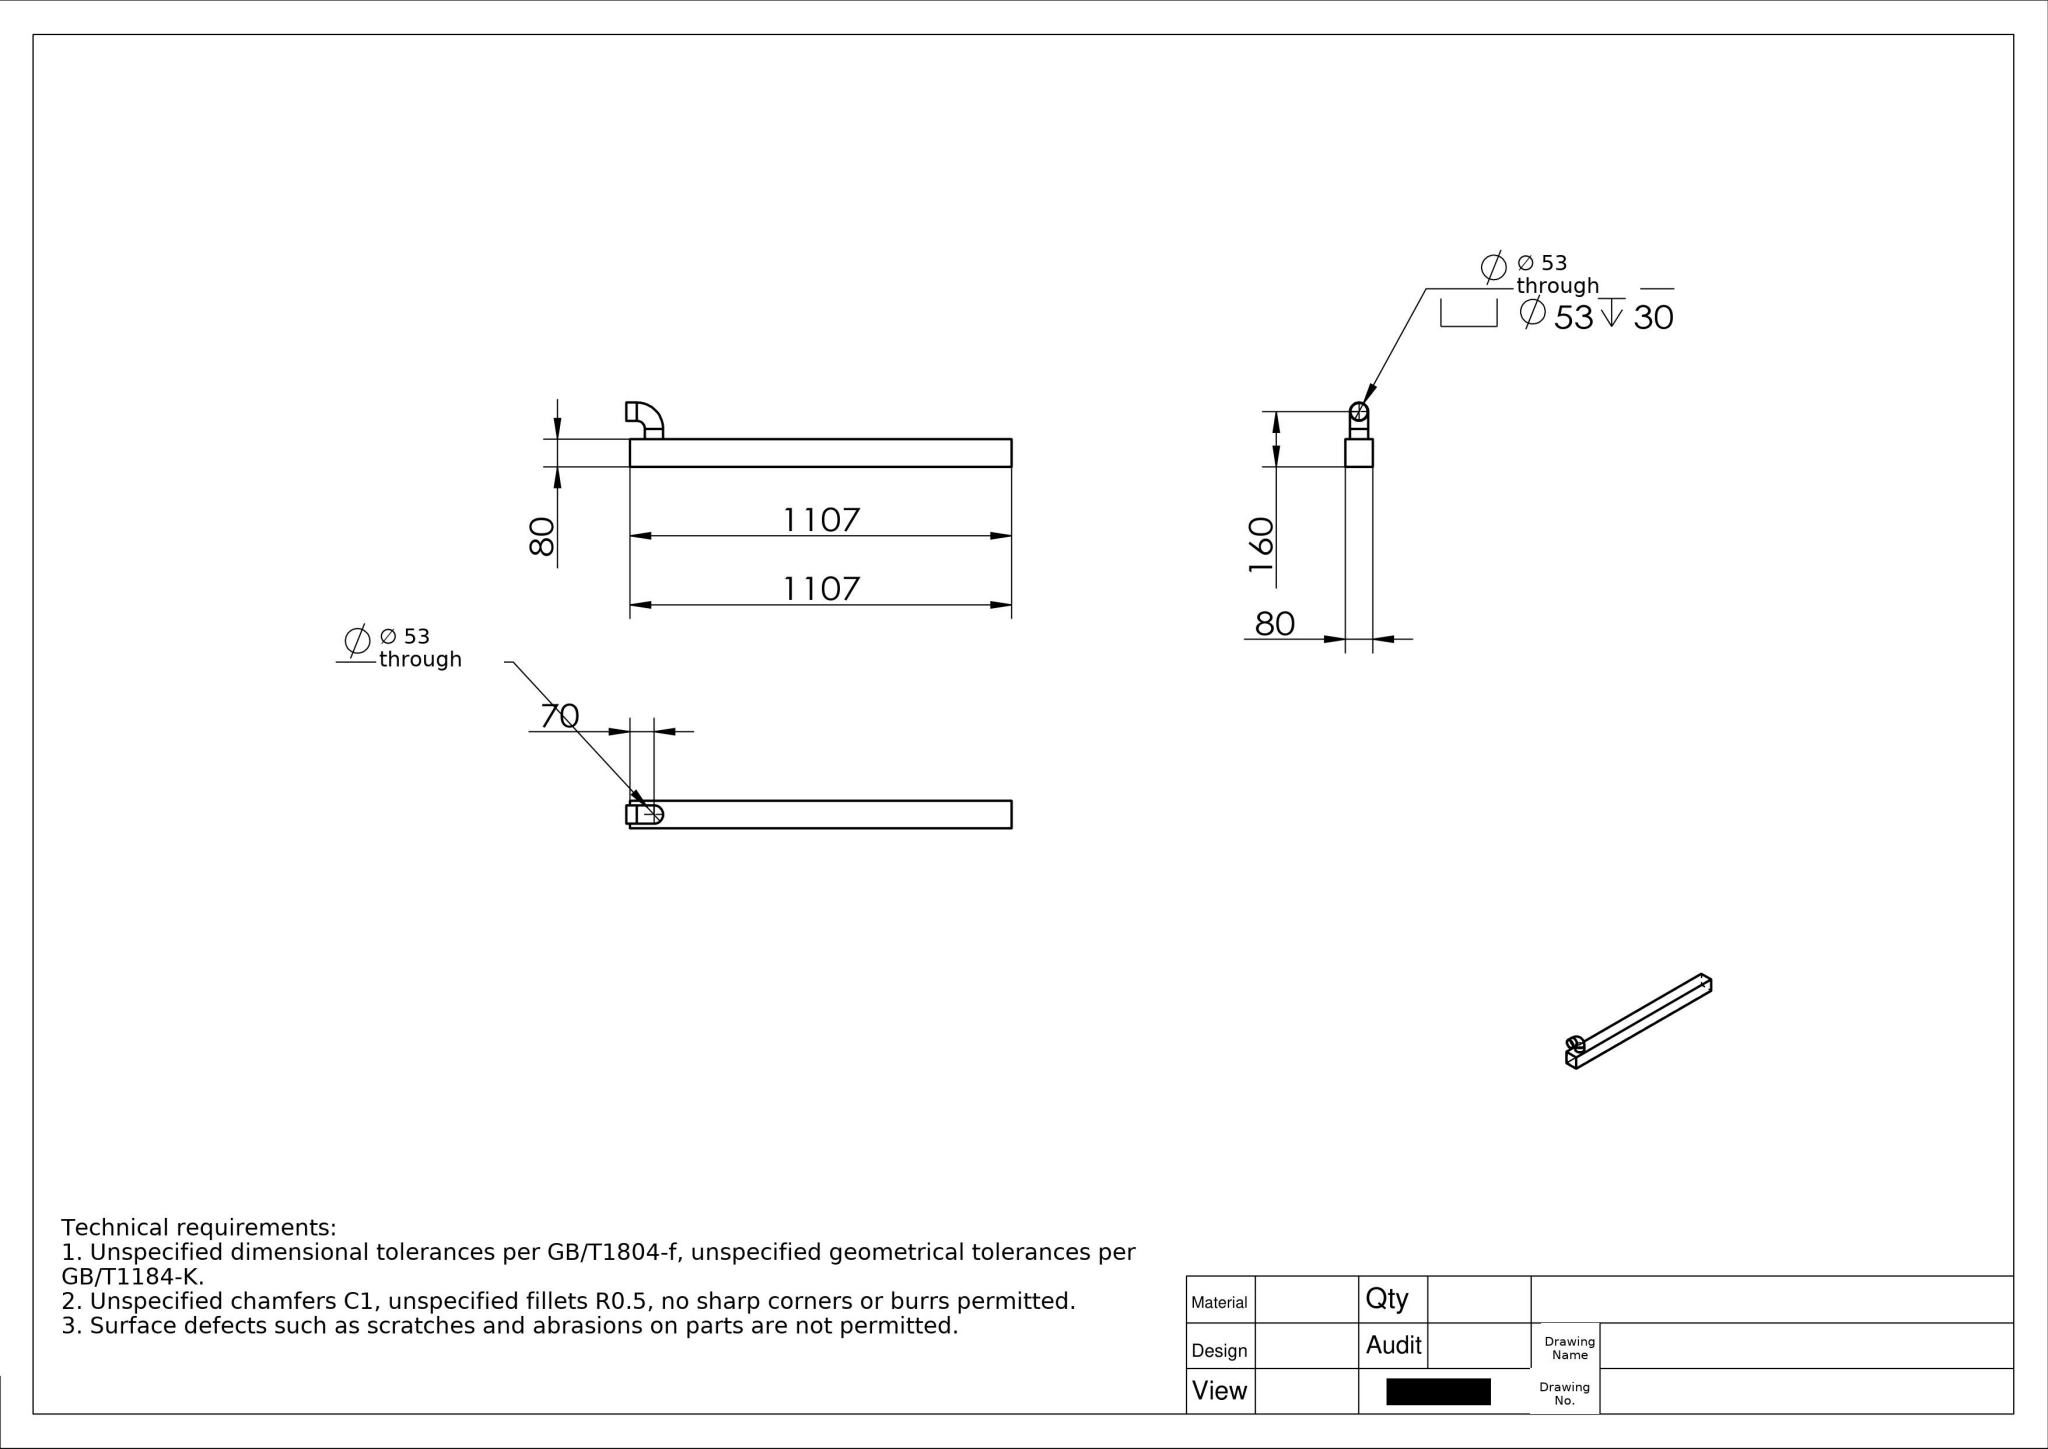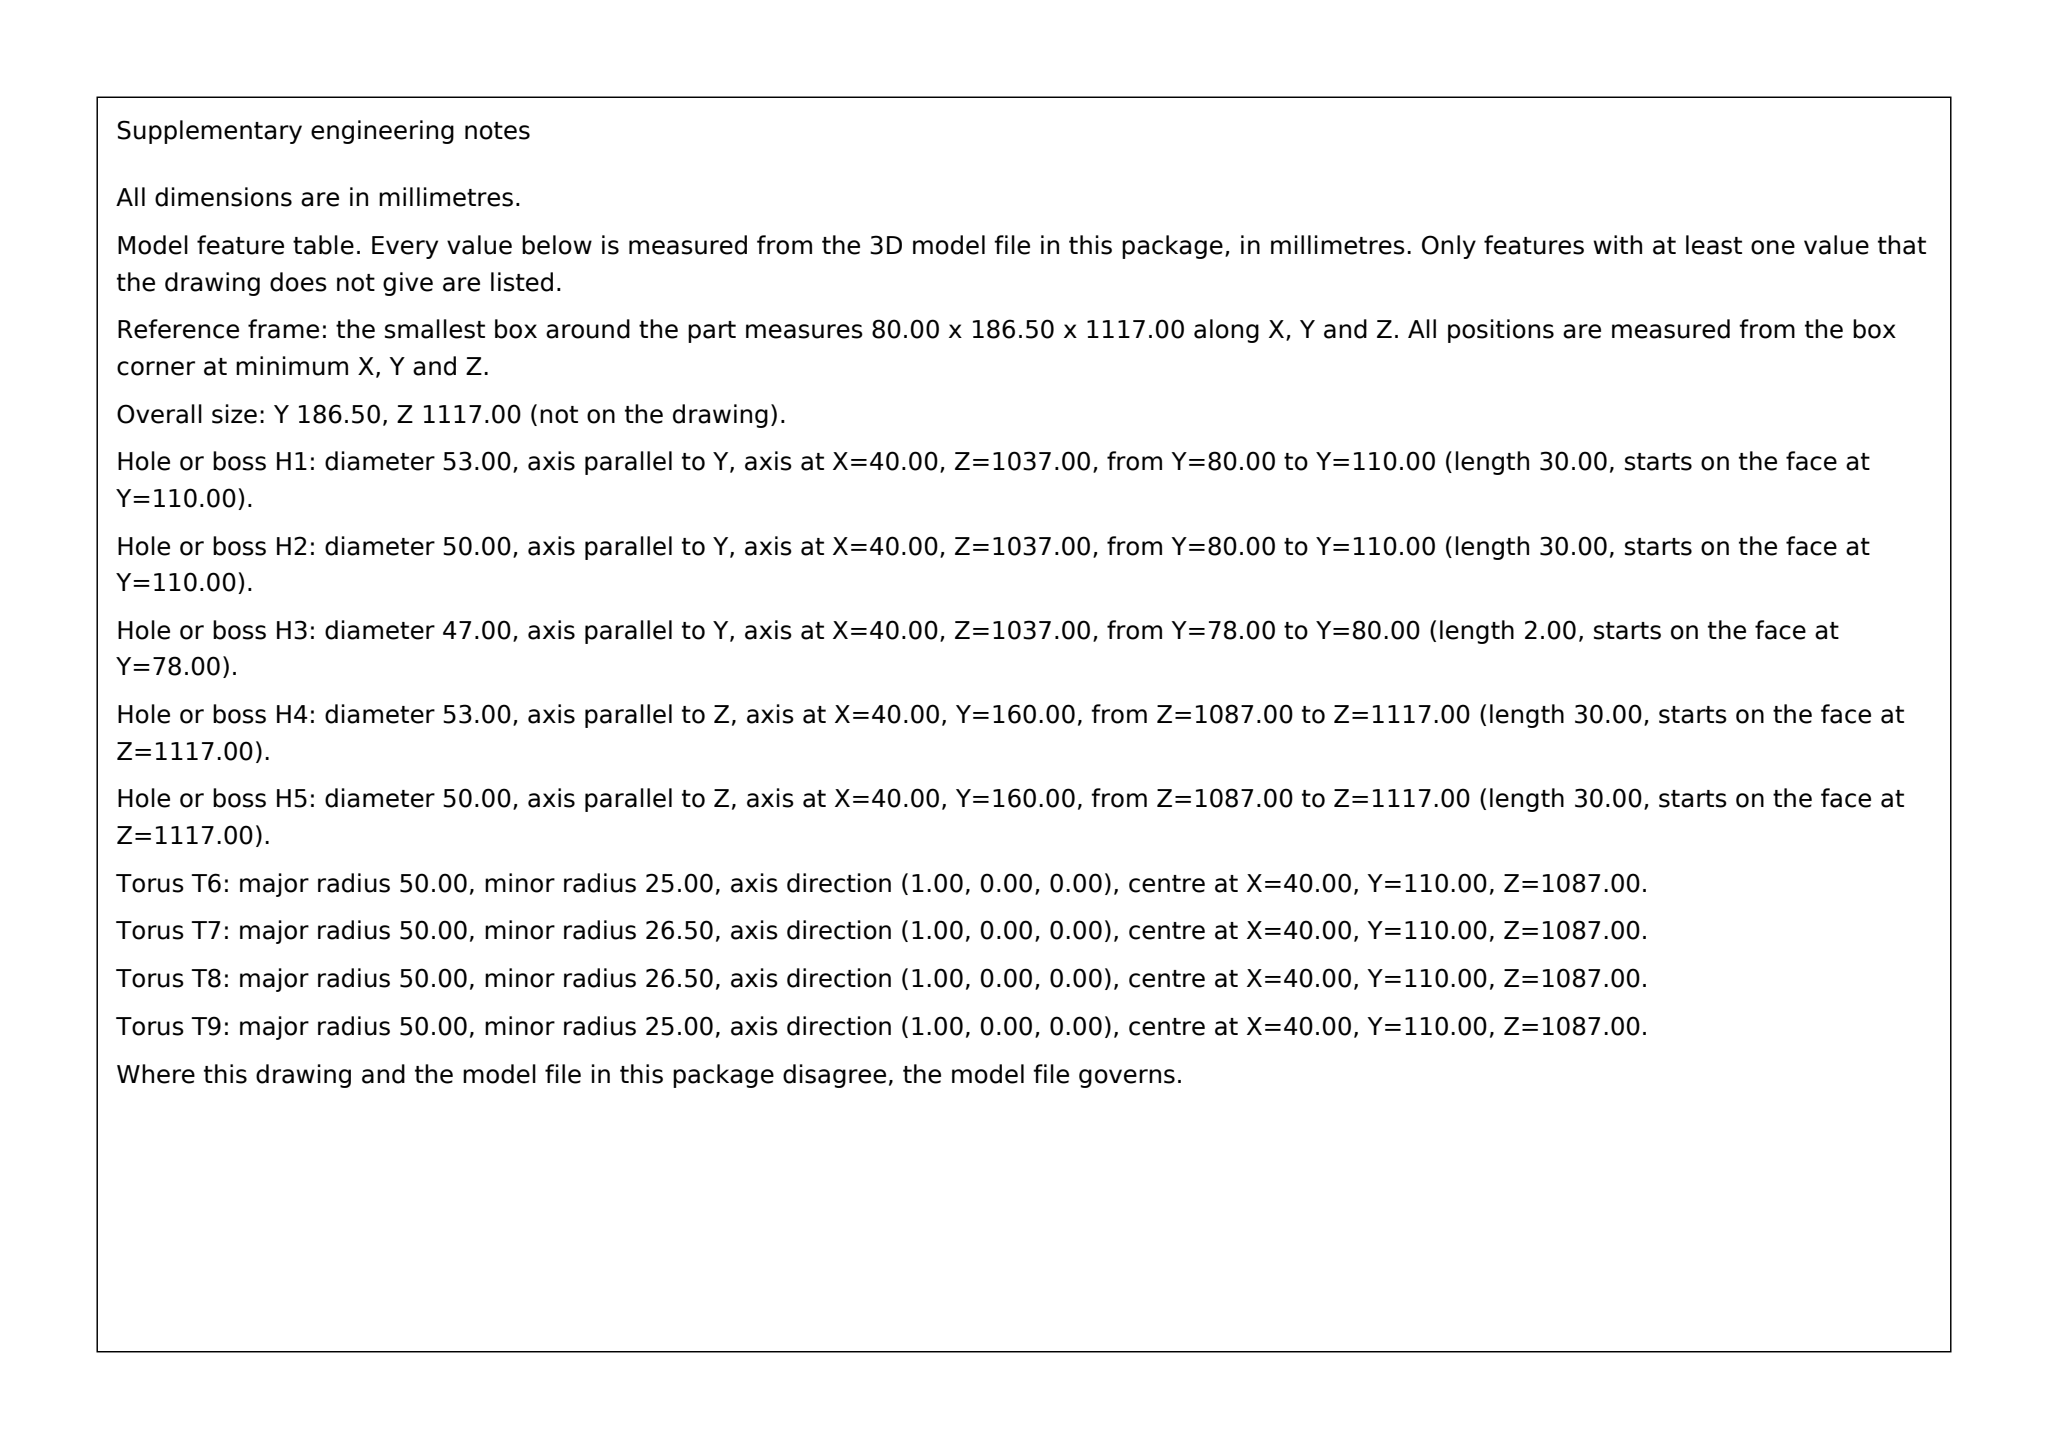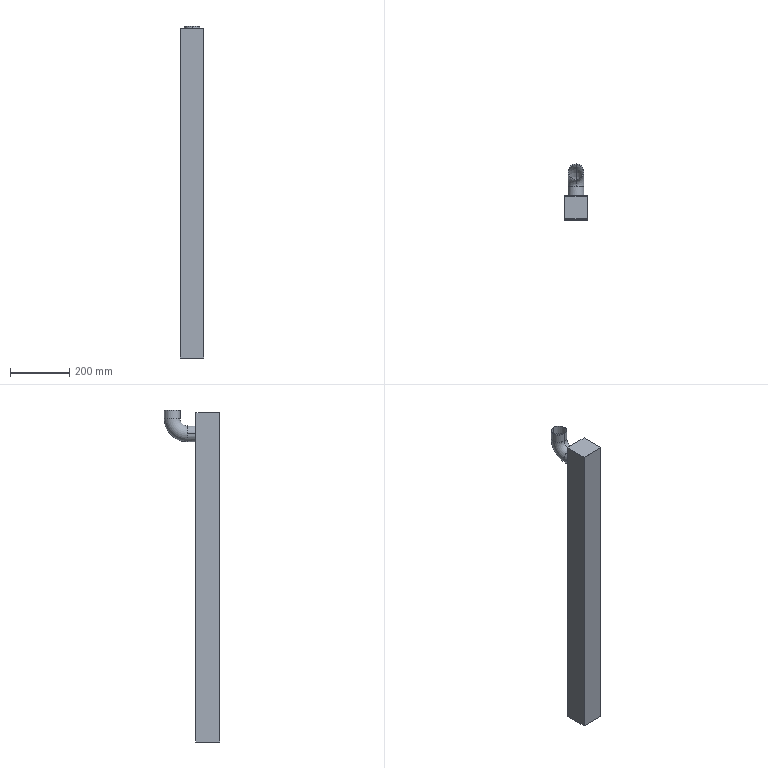Part | SolidWorks | mm | 1 solid | 27 faces | box 80 x 186.5 x 1117 mm | volume 738248 mm3 | plane 13 | cylinder 10 | torus 4 | commonest cylinder face diameters 50 x4 53 x4 47 x2
build123d program:
from build123d import *

# Parameters (mm, degrees)
SKETCH1_W                   = 80
SKETCH1_H                   = 80
SKETCH1_W_2                 = 76
SKETCH1_H_2                 = 76
BOSS_EXTRUDE1_DEPTH         = 1107
SKETCH2_W                   = 76
SKETCH2_H                   = 76
BOSS_EXTRUDE2_DEPTH         = 3
SKETCH3_R                   = 23.5
CUT_EXTRUDE1_DEPTH          = 10
SCAN_THIN_PART1_PROFILE_R   = 26.5
SCAN_THIN_PART1_PROFILE_R_2 = 25


with BuildPart() as part:
    # Sketch1 → Boss-Extrude1 (new body)
    with BuildSketch(Plane.XY):
        Rectangle(SKETCH1_W, SKETCH1_H)
        Rectangle(SKETCH1_W_2, SKETCH1_H_2, mode=Mode.SUBTRACT)
    extrude(amount=BOSS_EXTRUDE1_DEPTH)

    # Sketch2 → Boss-Extrude2 (add)
    with BuildSketch(Plane.XY.offset(1107)):
        Rectangle(SKETCH2_W, SKETCH2_H)
    extrude(amount=-BOSS_EXTRUDE2_DEPTH)

    # Sketch3 → Cut-Extrude1 (cut)
    with BuildSketch(Plane(origin=(0, 40, 0), x_dir=(1, 0, 0), z_dir=(0, 1, 0))):
        with Locations(Location((0, -1037, 0), (0, 0, 270))):
            Circle(SKETCH3_R)
    extrude(amount=-CUT_EXTRUDE1_DEPTH, mode=Mode.SUBTRACT)

    # Scan-Thin Part1: sweep along a path in Sketch4
    with BuildLine(Plane(origin=(0, 0, 0), x_dir=(0, 0, -1), z_dir=(1, 0, 0))) as scan_thin_part1_path:
        Line((-1037, 40), (-1037, 70))
        ThreePointArc((-1037, 70), (-1051.645, 105.355), (-1087, 120))
        Line((-1087, 120), (-1117, 120))
    # Scan-Thin Part1 profile (on start of the path) → Scan-Thin Part1 (sweep)
    with BuildSketch(Plane(origin=(0, 40, 1037), x_dir=(1, 0, 0), z_dir=(0, 1, 0))):
        Circle(SCAN_THIN_PART1_PROFILE_R)
        Circle(SCAN_THIN_PART1_PROFILE_R_2, mode=Mode.SUBTRACT)
    sweep(path=scan_thin_part1_path.line)


solid = part.part
STEP:
#1=CARTESIAN_POINT('',(-25.,70.,1037.));
#2=VERTEX_POINT('',#1);
#3=CARTESIAN_POINT('',(-0.,70.,1012.));
#4=VERTEX_POINT('',#3);
#5=CARTESIAN_POINT('',(-0.,70.,1037.));
#6=DIRECTION('',(0.,-1.,0.));
#7=DIRECTION('',(-1.,0.,0.));
#8=AXIS2_PLACEMENT_3D('',#5,#6,#7);
#9=CIRCLE('',#8,25.);
#10=EDGE_CURVE('',#2,#4,#9,.T.);
#11=ORIENTED_EDGE('',*,*,#10,.T.);
#12=CARTESIAN_POINT('',(-0.,145.,1087.));
#13=VERTEX_POINT('',#12);
#14=CARTESIAN_POINT('',(-0.,70.,1087.));
#15=DIRECTION('',(1.,0.,0.));
#16=DIRECTION('',(-0.,1.,0.));
#17=AXIS2_PLACEMENT_3D('',#14,#15,#16);
#18=CIRCLE('',#17,75.);
#19=EDGE_CURVE('',#4,#13,#18,.T.);
#20=ORIENTED_EDGE('',*,*,#19,.T.);
#21=CARTESIAN_POINT('',(-0.,95.,1087.));
#22=VERTEX_POINT('',#21);
#23=CARTESIAN_POINT('',(-0.,120.,1087.));
#24=DIRECTION('',(0.,0.,-1.));
#25=DIRECTION('',(-1.,0.,0.));
#26=AXIS2_PLACEMENT_3D('',#23,#24,#25);
#27=CIRCLE('',#26,25.);
#28=EDGE_CURVE('',#22,#13,#27,.T.);
#29=ORIENTED_EDGE('',*,*,#28,.F.);
#30=CARTESIAN_POINT('',(-0.,70.,1062.));
#31=VERTEX_POINT('',#30);
#32=CARTESIAN_POINT('',(-0.,70.,1087.));
#33=DIRECTION('',(1.,0.,0.));
#34=DIRECTION('',(-0.,1.,0.));
#35=AXIS2_PLACEMENT_3D('',#32,#33,#34);
#36=CIRCLE('',#35,25.);
#37=EDGE_CURVE('',#31,#22,#36,.T.);
#38=ORIENTED_EDGE('',*,*,#37,.F.);
#39=CARTESIAN_POINT('',(-0.,70.,1037.));
#40=DIRECTION('',(0.,-1.,0.));
#41=DIRECTION('',(-1.,0.,0.));
#42=AXIS2_PLACEMENT_3D('',#39,#40,#41);
#43=CIRCLE('',#42,25.);
#44=EDGE_CURVE('',#31,#2,#43,.T.);
#45=ORIENTED_EDGE('',*,*,#44,.T.);
#46=EDGE_LOOP('',(#11,#20,#29,#38,#45));
#47=FACE_OUTER_BOUND('',#46,.T.);
#48=CARTESIAN_POINT('',(-0.,70.,1087.));
#49=DIRECTION('',(1.,0.,0.));
#50=DIRECTION('',(-0.,1.,0.));
#51=AXIS2_PLACEMENT_3D('',#48,#49,#50);
#52=TOROIDAL_SURFACE('',#51,50.,25.);
#53=ADVANCED_FACE('',(#47),#52,.F.);
#54=CARTESIAN_POINT('',(-0.,70.,1010.5));
#55=VERTEX_POINT('',#54);
#56=CARTESIAN_POINT('',(26.5,70.,1037.));
#57=VERTEX_POINT('',#56);
#58=CARTESIAN_POINT('',(-0.,70.,1037.));
#59=DIRECTION('',(0.,-1.,0.));
#60=DIRECTION('',(-1.,0.,0.));
#61=AXIS2_PLACEMENT_3D('',#58,#59,#60);
#62=CIRCLE('',#61,26.5);
#63=EDGE_CURVE('',#55,#57,#62,.T.);
#64=ORIENTED_EDGE('',*,*,#63,.F.);
#65=CARTESIAN_POINT('',(-0.,146.5,1087.));
#66=VERTEX_POINT('',#65);
#67=CARTESIAN_POINT('',(-0.,70.,1087.));
#68=DIRECTION('',(1.,0.,0.));
#69=DIRECTION('',(-0.,1.,0.));
#70=AXIS2_PLACEMENT_3D('',#67,#68,#69);
#71=CIRCLE('',#70,76.5);
#72=EDGE_CURVE('',#55,#66,#71,.T.);
#73=ORIENTED_EDGE('',*,*,#72,.T.);
#74=CARTESIAN_POINT('',(-0.,93.5,1087.));
#75=VERTEX_POINT('',#74);
#76=CARTESIAN_POINT('',(-0.,120.,1087.));
#77=DIRECTION('',(0.,0.,-1.));
#78=DIRECTION('',(-1.,0.,0.));
#79=AXIS2_PLACEMENT_3D('',#76,#77,#78);
#80=CIRCLE('',#79,26.5);
#81=EDGE_CURVE('',#66,#75,#80,.T.);
#82=ORIENTED_EDGE('',*,*,#81,.T.);
#83=CARTESIAN_POINT('',(-0.,70.,1063.5));
#84=VERTEX_POINT('',#83);
#85=CARTESIAN_POINT('',(-0.,70.,1087.));
#86=DIRECTION('',(1.,0.,0.));
#87=DIRECTION('',(-0.,1.,0.));
#88=AXIS2_PLACEMENT_3D('',#85,#86,#87);
#89=CIRCLE('',#88,23.5);
#90=EDGE_CURVE('',#84,#75,#89,.T.);
#91=ORIENTED_EDGE('',*,*,#90,.F.);
#92=CARTESIAN_POINT('',(-0.,70.,1037.));
#93=DIRECTION('',(0.,-1.,0.));
#94=DIRECTION('',(-1.,0.,0.));
#95=AXIS2_PLACEMENT_3D('',#92,#93,#94);
#96=CIRCLE('',#95,26.5);
#97=EDGE_CURVE('',#57,#84,#96,.T.);
#98=ORIENTED_EDGE('',*,*,#97,.F.);
#99=EDGE_LOOP('',(#64,#73,#82,#91,#98));
#100=FACE_OUTER_BOUND('',#99,.T.);
#101=CARTESIAN_POINT('',(-0.,70.,1087.));
#102=DIRECTION('',(1.,0.,0.));
#103=DIRECTION('',(-0.,1.,0.));
#104=AXIS2_PLACEMENT_3D('',#101,#102,#103);
#105=TOROIDAL_SURFACE('',#104,50.,26.5);
#106=ADVANCED_FACE('',(#100),#105,.T.);
#107=ORIENTED_EDGE('',*,*,#28,.T.);
#108=CARTESIAN_POINT('',(-0.,145.,1117.));
#109=VERTEX_POINT('',#108);
#110=CARTESIAN_POINT('',(-0.,145.,1087.));
#111=DIRECTION('',(0.,-0.,1.));
#112=VECTOR('',#111,1000.);
#113=LINE('',#110,#112);
#114=EDGE_CURVE('',#13,#109,#113,.T.);
#115=ORIENTED_EDGE('',*,*,#114,.T.);
#116=CARTESIAN_POINT('',(-0.,95.,1117.));
#117=VERTEX_POINT('',#116);
#118=CARTESIAN_POINT('',(-0.,120.,1117.));
#119=DIRECTION('',(0.,0.,-1.));
#120=DIRECTION('',(-1.,0.,0.));
#121=AXIS2_PLACEMENT_3D('',#118,#119,#120);
#122=CIRCLE('',#121,25.);
#123=EDGE_CURVE('',#117,#109,#122,.T.);
#124=ORIENTED_EDGE('',*,*,#123,.F.);
#125=CARTESIAN_POINT('',(-0.,95.,1087.));
#126=DIRECTION('',(0.,-0.,1.));
#127=VECTOR('',#126,1000.);
#128=LINE('',#125,#127);
#129=EDGE_CURVE('',#22,#117,#128,.T.);
#130=ORIENTED_EDGE('',*,*,#129,.F.);
#131=EDGE_LOOP('',(#107,#115,#124,#130));
#132=FACE_OUTER_BOUND('',#131,.T.);
#133=CARTESIAN_POINT('',(-0.,120.,1087.));
#134=DIRECTION('',(0.,-0.,1.));
#135=DIRECTION('',(0.,-1.,0.));
#136=AXIS2_PLACEMENT_3D('',#133,#134,#135);
#137=CYLINDRICAL_SURFACE('',#136,25.);
#138=ADVANCED_FACE('',(#132),#137,.F.);
#139=CARTESIAN_POINT('',(-25.,40.,1037.));
#140=VERTEX_POINT('',#139);
#141=CARTESIAN_POINT('',(25.,40.,1037.));
#142=VERTEX_POINT('',#141);
#143=CARTESIAN_POINT('',(-0.,40.,1037.));
#144=DIRECTION('',(0.,-1.,0.));
#145=DIRECTION('',(-1.,-0.,0.));
#146=AXIS2_PLACEMENT_3D('',#143,#144,#145);
#147=CIRCLE('',#146,25.);
#148=EDGE_CURVE('',#140,#142,#147,.T.);
#149=ORIENTED_EDGE('',*,*,#148,.T.);
#150=CARTESIAN_POINT('',(25.,70.,1037.));
#151=VERTEX_POINT('',#150);
#152=CARTESIAN_POINT('',(25.,40.,1037.));
#153=DIRECTION('',(-0.,1.,0.));
#154=VECTOR('',#153,1000.);
#155=LINE('',#152,#154);
#156=EDGE_CURVE('',#142,#151,#155,.T.);
#157=ORIENTED_EDGE('',*,*,#156,.T.);
#158=CARTESIAN_POINT('',(-0.,70.,1037.));
#159=DIRECTION('',(0.,-1.,0.));
#160=DIRECTION('',(-1.,0.,0.));
#161=AXIS2_PLACEMENT_3D('',#158,#159,#160);
#162=CIRCLE('',#161,25.);
#163=EDGE_CURVE('',#4,#151,#162,.T.);
#164=ORIENTED_EDGE('',*,*,#163,.F.);
#165=ORIENTED_EDGE('',*,*,#10,.F.);
#166=CARTESIAN_POINT('',(-25.,40.,1037.));
#167=DIRECTION('',(-0.,1.,0.));
#168=VECTOR('',#167,1000.);
#169=LINE('',#166,#168);
#170=EDGE_CURVE('',#140,#2,#169,.T.);
#171=ORIENTED_EDGE('',*,*,#170,.F.);
#172=EDGE_LOOP('',(#149,#157,#164,#165,#171));
#173=FACE_OUTER_BOUND('',#172,.T.);
#174=CARTESIAN_POINT('',(-0.,40.,1037.));
#175=DIRECTION('',(-0.,1.,0.));
#176=DIRECTION('',(-1.,-0.,0.));
#177=AXIS2_PLACEMENT_3D('',#174,#175,#176);
#178=CYLINDRICAL_SURFACE('',#177,25.);
#179=ADVANCED_FACE('',(#173),#178,.F.);
#180=ORIENTED_EDGE('',*,*,#81,.F.);
#181=CARTESIAN_POINT('',(-0.,146.5,1117.));
#182=VERTEX_POINT('',#181);
#183=CARTESIAN_POINT('',(-0.,146.5,1087.));
#184=DIRECTION('',(0.,-0.,1.));
#185=VECTOR('',#184,1000.);
#186=LINE('',#183,#185);
#187=EDGE_CURVE('',#66,#182,#186,.T.);
#188=ORIENTED_EDGE('',*,*,#187,.T.);
#189=CARTESIAN_POINT('',(-0.,93.5,1117.));
#190=VERTEX_POINT('',#189);
#191=CARTESIAN_POINT('',(-0.,120.,1117.));
#192=DIRECTION('',(0.,0.,-1.));
#193=DIRECTION('',(-1.,0.,0.));
#194=AXIS2_PLACEMENT_3D('',#191,#192,#193);
#195=CIRCLE('',#194,26.5);
#196=EDGE_CURVE('',#182,#190,#195,.T.);
#197=ORIENTED_EDGE('',*,*,#196,.T.);
#198=CARTESIAN_POINT('',(-0.,93.5,1087.));
#199=DIRECTION('',(0.,-0.,1.));
#200=VECTOR('',#199,1000.);
#201=LINE('',#198,#200);
#202=EDGE_CURVE('',#75,#190,#201,.T.);
#203=ORIENTED_EDGE('',*,*,#202,.F.);
#204=EDGE_LOOP('',(#180,#188,#197,#203));
#205=FACE_OUTER_BOUND('',#204,.T.);
#206=CARTESIAN_POINT('',(-0.,120.,1087.));
#207=DIRECTION('',(0.,-0.,1.));
#208=DIRECTION('',(0.,-1.,0.));
#209=AXIS2_PLACEMENT_3D('',#206,#207,#208);
#210=CYLINDRICAL_SURFACE('',#209,26.5);
#211=ADVANCED_FACE('',(#205),#210,.T.);
#212=CARTESIAN_POINT('',(-26.5,40.,1037.));
#213=VERTEX_POINT('',#212);
#214=CARTESIAN_POINT('',(26.5,40.,1037.));
#215=VERTEX_POINT('',#214);
#216=CARTESIAN_POINT('',(-0.,40.,1037.));
#217=DIRECTION('',(0.,1.,0.));
#218=DIRECTION('',(0.,0.,-1.));
#219=AXIS2_PLACEMENT_3D('',#216,#217,#218);
#220=CIRCLE('',#219,26.5);
#221=EDGE_CURVE('',#213,#215,#220,.T.);
#222=ORIENTED_EDGE('',*,*,#221,.T.);
#223=CARTESIAN_POINT('',(26.5,40.,1037.));
#224=DIRECTION('',(-0.,1.,0.));
#225=VECTOR('',#224,1000.);
#226=LINE('',#223,#225);
#227=EDGE_CURVE('',#215,#57,#226,.T.);
#228=ORIENTED_EDGE('',*,*,#227,.T.);
#229=ORIENTED_EDGE('',*,*,#97,.T.);
#230=CARTESIAN_POINT('',(-26.5,70.,1037.));
#231=VERTEX_POINT('',#230);
#232=CARTESIAN_POINT('',(-0.,70.,1037.));
#233=DIRECTION('',(0.,-1.,0.));
#234=DIRECTION('',(-1.,0.,0.));
#235=AXIS2_PLACEMENT_3D('',#232,#233,#234);
#236=CIRCLE('',#235,26.5);
#237=EDGE_CURVE('',#84,#231,#236,.T.);
#238=ORIENTED_EDGE('',*,*,#237,.T.);
#239=CARTESIAN_POINT('',(-26.5,40.,1037.));
#240=DIRECTION('',(-0.,1.,0.));
#241=VECTOR('',#240,1000.);
#242=LINE('',#239,#241);
#243=EDGE_CURVE('',#213,#231,#242,.T.);
#244=ORIENTED_EDGE('',*,*,#243,.F.);
#245=EDGE_LOOP('',(#222,#228,#229,#238,#244));
#246=FACE_OUTER_BOUND('',#245,.T.);
#247=CARTESIAN_POINT('',(-0.,40.,1037.));
#248=DIRECTION('',(-0.,1.,0.));
#249=DIRECTION('',(-1.,-0.,0.));
#250=AXIS2_PLACEMENT_3D('',#247,#248,#249);
#251=CYLINDRICAL_SURFACE('',#250,26.5);
#252=ADVANCED_FACE('',(#246),#251,.T.);
#253=CARTESIAN_POINT('',(0.,38.,1060.5));
#254=VERTEX_POINT('',#253);
#255=CARTESIAN_POINT('',(0.,38.,1013.5));
#256=VERTEX_POINT('',#255);
#257=CARTESIAN_POINT('',(0.,38.,1037.));
#258=DIRECTION('',(0.,-1.,0.));
#259=DIRECTION('',(0.,0.,-1.));
#260=AXIS2_PLACEMENT_3D('',#257,#258,#259);
#261=CIRCLE('',#260,23.5);
#262=EDGE_CURVE('',#254,#256,#261,.T.);
#263=ORIENTED_EDGE('',*,*,#262,.T.);
#264=CARTESIAN_POINT('',(0.,40.,1013.5));
#265=VERTEX_POINT('',#264);
#266=CARTESIAN_POINT('',(0.,30.,1013.5));
#267=DIRECTION('',(0.,1.,0.));
#268=VECTOR('',#267,1000.);
#269=LINE('',#266,#268);
#270=EDGE_CURVE('',#256,#265,#269,.T.);
#271=ORIENTED_EDGE('',*,*,#270,.T.);
#272=CARTESIAN_POINT('',(0.,40.,1060.5));
#273=VERTEX_POINT('',#272);
#274=CARTESIAN_POINT('',(0.,40.,1037.));
#275=DIRECTION('',(0.,1.,0.));
#276=DIRECTION('',(0.,0.,1.));
#277=AXIS2_PLACEMENT_3D('',#274,#275,#276);
#278=CIRCLE('',#277,23.5);
#279=EDGE_CURVE('',#265,#273,#278,.T.);
#280=ORIENTED_EDGE('',*,*,#279,.T.);
#281=CARTESIAN_POINT('',(0.,30.,1060.5));
#282=DIRECTION('',(0.,1.,0.));
#283=VECTOR('',#282,1000.);
#284=LINE('',#281,#283);
#285=EDGE_CURVE('',#254,#273,#284,.T.);
#286=ORIENTED_EDGE('',*,*,#285,.F.);
#287=EDGE_LOOP('',(#263,#271,#280,#286));
#288=FACE_OUTER_BOUND('',#287,.T.);
#289=CARTESIAN_POINT('',(0.,30.,1037.));
#290=DIRECTION('',(0.,1.,0.));
#291=DIRECTION('',(0.,0.,1.));
#292=AXIS2_PLACEMENT_3D('',#289,#290,#291);
#293=CYLINDRICAL_SURFACE('',#292,23.5);
#294=ADVANCED_FACE('',(#288),#293,.F.);
#295=CARTESIAN_POINT('',(0.,40.,1037.));
#296=DIRECTION('',(0.,1.,0.));
#297=DIRECTION('',(0.,0.,1.));
#298=AXIS2_PLACEMENT_3D('',#295,#296,#297);
#299=CIRCLE('',#298,23.5);
#300=EDGE_CURVE('',#273,#265,#299,.T.);
#301=ORIENTED_EDGE('',*,*,#300,.F.);
#302=ORIENTED_EDGE('',*,*,#279,.F.);
#303=EDGE_LOOP('',(#301,#302));
#304=FACE_BOUND('',#303,.T.);
#305=ORIENTED_EDGE('',*,*,#148,.F.);
#306=CARTESIAN_POINT('',(-0.,40.,1037.));
#307=DIRECTION('',(0.,-1.,0.));
#308=DIRECTION('',(-1.,-0.,0.));
#309=AXIS2_PLACEMENT_3D('',#306,#307,#308);
#310=CIRCLE('',#309,25.);
#311=EDGE_CURVE('',#142,#140,#310,.T.);
#312=ORIENTED_EDGE('',*,*,#311,.F.);
#313=EDGE_LOOP('',(#305,#312));
#314=FACE_OUTER_BOUND('',#313,.T.);
#315=CARTESIAN_POINT('',(-40.,40.,1107.));
#316=DIRECTION('',(0.,-1.,0.));
#317=DIRECTION('',(0.,0.,-1.));
#318=AXIS2_PLACEMENT_3D('',#315,#316,#317);
#319=PLANE('',#318);
#320=ADVANCED_FACE('',(#304,#314),#319,.F.);
#321=CARTESIAN_POINT('',(38.,-38.,1104.));
#322=VERTEX_POINT('',#321);
#323=CARTESIAN_POINT('',(38.,-38.,0.));
#324=VERTEX_POINT('',#323);
#325=CARTESIAN_POINT('',(38.,-38.,1107.));
#326=DIRECTION('',(0.,0.,-1.));
#327=VECTOR('',#326,1000.);
#328=LINE('',#325,#327);
#329=EDGE_CURVE('',#322,#324,#328,.T.);
#330=ORIENTED_EDGE('',*,*,#329,.F.);
#331=CARTESIAN_POINT('',(38.,38.,1104.));
#332=VERTEX_POINT('',#331);
#333=CARTESIAN_POINT('',(38.,38.,1104.));
#334=DIRECTION('',(0.,1.,0.));
#335=VECTOR('',#334,1000.);
#336=LINE('',#333,#335);
#337=EDGE_CURVE('',#322,#332,#336,.T.);
#338=ORIENTED_EDGE('',*,*,#337,.T.);
#339=CARTESIAN_POINT('',(38.,38.,0.));
#340=VERTEX_POINT('',#339);
#341=CARTESIAN_POINT('',(38.,38.,1107.));
#342=DIRECTION('',(0.,0.,-1.));
#343=VECTOR('',#342,1000.);
#344=LINE('',#341,#343);
#345=EDGE_CURVE('',#332,#340,#344,.T.);
#346=ORIENTED_EDGE('',*,*,#345,.T.);
#347=CARTESIAN_POINT('',(38.,38.,0.));
#348=DIRECTION('',(-0.,1.,0.));
#349=VECTOR('',#348,1000.);
#350=LINE('',#347,#349);
#351=EDGE_CURVE('',#324,#340,#350,.T.);
#352=ORIENTED_EDGE('',*,*,#351,.F.);
#353=EDGE_LOOP('',(#330,#338,#346,#352));
#354=FACE_OUTER_BOUND('',#353,.T.);
#355=CARTESIAN_POINT('',(38.,38.,1107.));
#356=DIRECTION('',(-1.,-0.,0.));
#357=DIRECTION('',(0.,-1.,0.));
#358=AXIS2_PLACEMENT_3D('',#355,#356,#357);
#359=PLANE('',#358);
#360=ADVANCED_FACE('',(#354),#359,.T.);
#361=ORIENTED_EDGE('',*,*,#262,.F.);
#362=CARTESIAN_POINT('',(0.,38.,1037.));
#363=DIRECTION('',(0.,-1.,0.));
#364=DIRECTION('',(0.,0.,-1.));
#365=AXIS2_PLACEMENT_3D('',#362,#363,#364);
#366=CIRCLE('',#365,23.5);
#367=EDGE_CURVE('',#256,#254,#366,.T.);
#368=ORIENTED_EDGE('',*,*,#367,.F.);
#369=EDGE_LOOP('',(#361,#368));
#370=FACE_BOUND('',#369,.T.);
#371=ORIENTED_EDGE('',*,*,#345,.F.);
#372=CARTESIAN_POINT('',(-38.,38.,1104.));
#373=VERTEX_POINT('',#372);
#374=CARTESIAN_POINT('',(-38.,38.,1104.));
#375=DIRECTION('',(-1.,0.,0.));
#376=VECTOR('',#375,1000.);
#377=LINE('',#374,#376);
#378=EDGE_CURVE('',#332,#373,#377,.T.);
#379=ORIENTED_EDGE('',*,*,#378,.T.);
#380=CARTESIAN_POINT('',(-38.,38.,0.));
#381=VERTEX_POINT('',#380);
#382=CARTESIAN_POINT('',(-38.,38.,1107.));
#383=DIRECTION('',(0.,0.,-1.));
#384=VECTOR('',#383,1000.);
#385=LINE('',#382,#384);
#386=EDGE_CURVE('',#373,#381,#385,.T.);
#387=ORIENTED_EDGE('',*,*,#386,.T.);
#388=CARTESIAN_POINT('',(-38.,38.,0.));
#389=DIRECTION('',(-1.,0.,0.));
#390=VECTOR('',#389,1000.);
#391=LINE('',#388,#390);
#392=EDGE_CURVE('',#340,#381,#391,.T.);
#393=ORIENTED_EDGE('',*,*,#392,.F.);
#394=EDGE_LOOP('',(#371,#379,#387,#393));
#395=FACE_OUTER_BOUND('',#394,.T.);
#396=CARTESIAN_POINT('',(-38.,38.,1107.));
#397=DIRECTION('',(0.,-1.,0.));
#398=DIRECTION('',(0.,0.,-1.));
#399=AXIS2_PLACEMENT_3D('',#396,#397,#398);
#400=PLANE('',#399);
#401=ADVANCED_FACE('',(#370,#395),#400,.T.);
#402=ORIENTED_EDGE('',*,*,#386,.F.);
#403=CARTESIAN_POINT('',(-38.,-38.,1104.));
#404=VERTEX_POINT('',#403);
#405=CARTESIAN_POINT('',(-38.,38.,1104.));
#406=DIRECTION('',(0.,-1.,0.));
#407=VECTOR('',#406,1000.);
#408=LINE('',#405,#407);
#409=EDGE_CURVE('',#373,#404,#408,.T.);
#410=ORIENTED_EDGE('',*,*,#409,.T.);
#411=CARTESIAN_POINT('',(-38.,-38.,0.));
#412=VERTEX_POINT('',#411);
#413=CARTESIAN_POINT('',(-38.,-38.,1107.));
#414=DIRECTION('',(0.,0.,-1.));
#415=VECTOR('',#414,1000.);
#416=LINE('',#413,#415);
#417=EDGE_CURVE('',#404,#412,#416,.T.);
#418=ORIENTED_EDGE('',*,*,#417,.T.);
#419=CARTESIAN_POINT('',(-38.,38.,0.));
#420=DIRECTION('',(0.,-1.,0.));
#421=VECTOR('',#420,1000.);
#422=LINE('',#419,#421);
#423=EDGE_CURVE('',#381,#412,#422,.T.);
#424=ORIENTED_EDGE('',*,*,#423,.F.);
#425=EDGE_LOOP('',(#402,#410,#418,#424));
#426=FACE_OUTER_BOUND('',#425,.T.);
#427=CARTESIAN_POINT('',(-38.,38.,1107.));
#428=DIRECTION('',(1.,0.,0.));
#429=DIRECTION('',(-0.,1.,0.));
#430=AXIS2_PLACEMENT_3D('',#427,#428,#429);
#431=PLANE('',#430);
#432=ADVANCED_FACE('',(#426),#431,.T.);
#433=ORIENTED_EDGE('',*,*,#417,.F.);
#434=CARTESIAN_POINT('',(-38.,-38.,1104.));
#435=DIRECTION('',(1.,0.,0.));
#436=VECTOR('',#435,1000.);
#437=LINE('',#434,#436);
#438=EDGE_CURVE('',#404,#322,#437,.T.);
#439=ORIENTED_EDGE('',*,*,#438,.T.);
#440=ORIENTED_EDGE('',*,*,#329,.T.);
#441=CARTESIAN_POINT('',(-38.,-38.,0.));
#442=DIRECTION('',(1.,0.,0.));
#443=VECTOR('',#442,1000.);
#444=LINE('',#441,#443);
#445=EDGE_CURVE('',#412,#324,#444,.T.);
#446=ORIENTED_EDGE('',*,*,#445,.F.);
#447=EDGE_LOOP('',(#433,#439,#440,#446));
#448=FACE_OUTER_BOUND('',#447,.T.);
#449=CARTESIAN_POINT('',(-38.,-38.,1107.));
#450=DIRECTION('',(0.,1.,0.));
#451=DIRECTION('',(0.,0.,1.));
#452=AXIS2_PLACEMENT_3D('',#449,#450,#451);
#453=PLANE('',#452);
#454=ADVANCED_FACE('',(#448),#453,.T.);
#455=CARTESIAN_POINT('',(40.,-40.,1107.));
#456=VERTEX_POINT('',#455);
#457=CARTESIAN_POINT('',(40.,40.,1107.));
#458=VERTEX_POINT('',#457);
#459=CARTESIAN_POINT('',(40.,40.,1107.));
#460=DIRECTION('',(-0.,1.,0.));
#461=VECTOR('',#460,1000.);
#462=LINE('',#459,#461);
#463=EDGE_CURVE('',#456,#458,#462,.T.);
#464=ORIENTED_EDGE('',*,*,#463,.T.);
#465=CARTESIAN_POINT('',(-40.,40.,1107.));
#466=VERTEX_POINT('',#465);
#467=CARTESIAN_POINT('',(-40.,40.,1107.));
#468=DIRECTION('',(-1.,0.,0.));
#469=VECTOR('',#468,1000.);
#470=LINE('',#467,#469);
#471=EDGE_CURVE('',#458,#466,#470,.T.);
#472=ORIENTED_EDGE('',*,*,#471,.T.);
#473=CARTESIAN_POINT('',(-40.,-40.,1107.));
#474=VERTEX_POINT('',#473);
#475=CARTESIAN_POINT('',(-40.,40.,1107.));
#476=DIRECTION('',(0.,-1.,0.));
#477=VECTOR('',#476,1000.);
#478=LINE('',#475,#477);
#479=EDGE_CURVE('',#466,#474,#478,.T.);
#480=ORIENTED_EDGE('',*,*,#479,.T.);
#481=CARTESIAN_POINT('',(-40.,-40.,1107.));
#482=DIRECTION('',(1.,0.,0.));
#483=VECTOR('',#482,1000.);
#484=LINE('',#481,#483);
#485=EDGE_CURVE('',#474,#456,#484,.T.);
#486=ORIENTED_EDGE('',*,*,#485,.T.);
#487=EDGE_LOOP('',(#464,#472,#480,#486));
#488=FACE_OUTER_BOUND('',#487,.T.);
#489=CARTESIAN_POINT('',(0.,0.,1107.));
#490=DIRECTION('',(0.,0.,1.));
#491=DIRECTION('',(1.,0.,0.));
#492=AXIS2_PLACEMENT_3D('',#489,#490,#491);
#493=PLANE('',#492);
#494=ADVANCED_FACE('',(#488),#493,.T.);
#495=CARTESIAN_POINT('',(40.,-40.,0.));
#496=VERTEX_POINT('',#495);
#497=CARTESIAN_POINT('',(40.,40.,0.));
#498=VERTEX_POINT('',#497);
#499=CARTESIAN_POINT('',(40.,40.,0.));
#500=DIRECTION('',(-0.,1.,0.));
#501=VECTOR('',#500,1000.);
#502=LINE('',#499,#501);
#503=EDGE_CURVE('',#496,#498,#502,.T.);
#504=ORIENTED_EDGE('',*,*,#503,.F.);
#505=CARTESIAN_POINT('',(-40.,-40.,0.));
#506=VERTEX_POINT('',#505);
#507=CARTESIAN_POINT('',(-40.,-40.,0.));
#508=DIRECTION('',(1.,0.,0.));
#509=VECTOR('',#508,1000.);
#510=LINE('',#507,#509);
#511=EDGE_CURVE('',#506,#496,#510,.T.);
#512=ORIENTED_EDGE('',*,*,#511,.F.);
#513=CARTESIAN_POINT('',(-40.,40.,0.));
#514=VERTEX_POINT('',#513);
#515=CARTESIAN_POINT('',(-40.,40.,0.));
#516=DIRECTION('',(0.,-1.,0.));
#517=VECTOR('',#516,1000.);
#518=LINE('',#515,#517);
#519=EDGE_CURVE('',#514,#506,#518,.T.);
#520=ORIENTED_EDGE('',*,*,#519,.F.);
#521=CARTESIAN_POINT('',(-40.,40.,0.));
#522=DIRECTION('',(-1.,0.,0.));
#523=VECTOR('',#522,1000.);
#524=LINE('',#521,#523);
#525=EDGE_CURVE('',#498,#514,#524,.T.);
#526=ORIENTED_EDGE('',*,*,#525,.F.);
#527=EDGE_LOOP('',(#504,#512,#520,#526));
#528=FACE_OUTER_BOUND('',#527,.T.);
#529=ORIENTED_EDGE('',*,*,#351,.T.);
#530=ORIENTED_EDGE('',*,*,#392,.T.);
#531=ORIENTED_EDGE('',*,*,#423,.T.);
#532=ORIENTED_EDGE('',*,*,#445,.T.);
#533=EDGE_LOOP('',(#529,#530,#531,#532));
#534=FACE_BOUND('',#533,.T.);
#535=CARTESIAN_POINT('',(0.,0.,0.));
#536=DIRECTION('',(0.,0.,1.));
#537=DIRECTION('',(1.,0.,0.));
#538=AXIS2_PLACEMENT_3D('',#535,#536,#537);
#539=PLANE('',#538);
#540=ADVANCED_FACE('',(#528,#534),#539,.F.);
#541=ORIENTED_EDGE('',*,*,#503,.T.);
#542=CARTESIAN_POINT('',(40.,40.,1107.));
#543=DIRECTION('',(0.,0.,-1.));
#544=VECTOR('',#543,1000.);
#545=LINE('',#542,#544);
#546=EDGE_CURVE('',#458,#498,#545,.T.);
#547=ORIENTED_EDGE('',*,*,#546,.F.);
#548=ORIENTED_EDGE('',*,*,#463,.F.);
#549=CARTESIAN_POINT('',(40.,-40.,1107.));
#550=DIRECTION('',(0.,0.,-1.));
#551=VECTOR('',#550,1000.);
#552=LINE('',#549,#551);
#553=EDGE_CURVE('',#456,#496,#552,.T.);
#554=ORIENTED_EDGE('',*,*,#553,.T.);
#555=EDGE_LOOP('',(#541,#547,#548,#554));
#556=FACE_OUTER_BOUND('',#555,.T.);
#557=CARTESIAN_POINT('',(40.,40.,1107.));
#558=DIRECTION('',(-1.,-0.,0.));
#559=DIRECTION('',(0.,-1.,0.));
#560=AXIS2_PLACEMENT_3D('',#557,#558,#559);
#561=PLANE('',#560);
#562=ADVANCED_FACE('',(#556),#561,.F.);
#563=ORIENTED_EDGE('',*,*,#221,.F.);
#564=CARTESIAN_POINT('',(-0.,40.,1037.));
#565=DIRECTION('',(0.,1.,0.));
#566=DIRECTION('',(0.,0.,-1.));
#567=AXIS2_PLACEMENT_3D('',#564,#565,#566);
#568=CIRCLE('',#567,26.5);
#569=EDGE_CURVE('',#215,#213,#568,.T.);
#570=ORIENTED_EDGE('',*,*,#569,.F.);
#571=EDGE_LOOP('',(#563,#570));
#572=FACE_BOUND('',#571,.T.);
#573=ORIENTED_EDGE('',*,*,#525,.T.);
#574=CARTESIAN_POINT('',(-40.,40.,1107.));
#575=DIRECTION('',(0.,0.,-1.));
#576=VECTOR('',#575,1000.);
#577=LINE('',#574,#576);
#578=EDGE_CURVE('',#466,#514,#577,.T.);
#579=ORIENTED_EDGE('',*,*,#578,.F.);
#580=ORIENTED_EDGE('',*,*,#471,.F.);
#581=ORIENTED_EDGE('',*,*,#546,.T.);
#582=EDGE_LOOP('',(#573,#579,#580,#581));
#583=FACE_OUTER_BOUND('',#582,.T.);
#584=CARTESIAN_POINT('',(-40.,40.,1107.));
#585=DIRECTION('',(0.,-1.,0.));
#586=DIRECTION('',(0.,0.,-1.));
#587=AXIS2_PLACEMENT_3D('',#584,#585,#586);
#588=PLANE('',#587);
#589=ADVANCED_FACE('',(#572,#583),#588,.F.);
#590=ORIENTED_EDGE('',*,*,#519,.T.);
#591=CARTESIAN_POINT('',(-40.,-40.,1107.));
#592=DIRECTION('',(0.,0.,-1.));
#593=VECTOR('',#592,1000.);
#594=LINE('',#591,#593);
#595=EDGE_CURVE('',#474,#506,#594,.T.);
#596=ORIENTED_EDGE('',*,*,#595,.F.);
#597=ORIENTED_EDGE('',*,*,#479,.F.);
#598=ORIENTED_EDGE('',*,*,#578,.T.);
#599=EDGE_LOOP('',(#590,#596,#597,#598));
#600=FACE_OUTER_BOUND('',#599,.T.);
#601=CARTESIAN_POINT('',(-40.,40.,1107.));
#602=DIRECTION('',(1.,0.,0.));
#603=DIRECTION('',(-0.,1.,0.));
#604=AXIS2_PLACEMENT_3D('',#601,#602,#603);
#605=PLANE('',#604);
#606=ADVANCED_FACE('',(#600),#605,.F.);
#607=ORIENTED_EDGE('',*,*,#511,.T.);
#608=ORIENTED_EDGE('',*,*,#553,.F.);
#609=ORIENTED_EDGE('',*,*,#485,.F.);
#610=ORIENTED_EDGE('',*,*,#595,.T.);
#611=EDGE_LOOP('',(#607,#608,#609,#610));
#612=FACE_OUTER_BOUND('',#611,.T.);
#613=CARTESIAN_POINT('',(-40.,-40.,1107.));
#614=DIRECTION('',(0.,1.,0.));
#615=DIRECTION('',(0.,0.,1.));
#616=AXIS2_PLACEMENT_3D('',#613,#614,#615);
#617=PLANE('',#616);
#618=ADVANCED_FACE('',(#612),#617,.F.);
#619=ORIENTED_EDGE('',*,*,#409,.F.);
#620=ORIENTED_EDGE('',*,*,#378,.F.);
#621=ORIENTED_EDGE('',*,*,#337,.F.);
#622=ORIENTED_EDGE('',*,*,#438,.F.);
#623=EDGE_LOOP('',(#619,#620,#621,#622));
#624=FACE_OUTER_BOUND('',#623,.T.);
#625=CARTESIAN_POINT('',(0.,0.,1104.));
#626=DIRECTION('',(0.,0.,1.));
#627=DIRECTION('',(1.,0.,0.));
#628=AXIS2_PLACEMENT_3D('',#625,#626,#627);
#629=PLANE('',#628);
#630=ADVANCED_FACE('',(#624),#629,.F.);
#631=ORIENTED_EDGE('',*,*,#270,.F.);
#632=ORIENTED_EDGE('',*,*,#367,.T.);
#633=ORIENTED_EDGE('',*,*,#285,.T.);
#634=ORIENTED_EDGE('',*,*,#300,.T.);
#635=EDGE_LOOP('',(#631,#632,#633,#634));
#636=FACE_OUTER_BOUND('',#635,.T.);
#637=CARTESIAN_POINT('',(0.,30.,1037.));
#638=DIRECTION('',(0.,1.,0.));
#639=DIRECTION('',(0.,0.,1.));
#640=AXIS2_PLACEMENT_3D('',#637,#638,#639);
#641=CYLINDRICAL_SURFACE('',#640,23.5);
#642=ADVANCED_FACE('',(#636),#641,.F.);
#643=ORIENTED_EDGE('',*,*,#187,.F.);
#644=CARTESIAN_POINT('',(-0.,120.,1087.));
#645=DIRECTION('',(0.,0.,-1.));
#646=DIRECTION('',(-1.,0.,0.));
#647=AXIS2_PLACEMENT_3D('',#644,#645,#646);
#648=CIRCLE('',#647,26.5);
#649=EDGE_CURVE('',#75,#66,#648,.T.);
#650=ORIENTED_EDGE('',*,*,#649,.F.);
#651=ORIENTED_EDGE('',*,*,#202,.T.);
#652=CARTESIAN_POINT('',(-0.,120.,1117.));
#653=DIRECTION('',(0.,0.,-1.));
#654=DIRECTION('',(-1.,0.,0.));
#655=AXIS2_PLACEMENT_3D('',#652,#653,#654);
#656=CIRCLE('',#655,26.5);
#657=EDGE_CURVE('',#190,#182,#656,.T.);
#658=ORIENTED_EDGE('',*,*,#657,.T.);
#659=EDGE_LOOP('',(#643,#650,#651,#658));
#660=FACE_OUTER_BOUND('',#659,.T.);
#661=CARTESIAN_POINT('',(-0.,120.,1087.));
#662=DIRECTION('',(0.,-0.,1.));
#663=DIRECTION('',(0.,-1.,0.));
#664=AXIS2_PLACEMENT_3D('',#661,#662,#663);
#665=CYLINDRICAL_SURFACE('',#664,26.5);
#666=ADVANCED_FACE('',(#660),#665,.T.);
#667=ORIENTED_EDGE('',*,*,#72,.F.);
#668=CARTESIAN_POINT('',(-0.,70.,1037.));
#669=DIRECTION('',(0.,-1.,0.));
#670=DIRECTION('',(-1.,0.,0.));
#671=AXIS2_PLACEMENT_3D('',#668,#669,#670);
#672=CIRCLE('',#671,26.5);
#673=EDGE_CURVE('',#231,#55,#672,.T.);
#674=ORIENTED_EDGE('',*,*,#673,.F.);
#675=ORIENTED_EDGE('',*,*,#237,.F.);
#676=ORIENTED_EDGE('',*,*,#90,.T.);
#677=ORIENTED_EDGE('',*,*,#649,.T.);
#678=EDGE_LOOP('',(#667,#674,#675,#676,#677));
#679=FACE_OUTER_BOUND('',#678,.T.);
#680=CARTESIAN_POINT('',(-0.,70.,1087.));
#681=DIRECTION('',(1.,0.,0.));
#682=DIRECTION('',(-0.,1.,0.));
#683=AXIS2_PLACEMENT_3D('',#680,#681,#682);
#684=TOROIDAL_SURFACE('',#683,50.,26.5);
#685=ADVANCED_FACE('',(#679),#684,.T.);
#686=ORIENTED_EDGE('',*,*,#227,.F.);
#687=ORIENTED_EDGE('',*,*,#569,.T.);
#688=ORIENTED_EDGE('',*,*,#243,.T.);
#689=ORIENTED_EDGE('',*,*,#673,.T.);
#690=ORIENTED_EDGE('',*,*,#63,.T.);
#691=EDGE_LOOP('',(#686,#687,#688,#689,#690));
#692=FACE_OUTER_BOUND('',#691,.T.);
#693=CARTESIAN_POINT('',(-0.,40.,1037.));
#694=DIRECTION('',(-0.,1.,0.));
#695=DIRECTION('',(-1.,-0.,0.));
#696=AXIS2_PLACEMENT_3D('',#693,#694,#695);
#697=CYLINDRICAL_SURFACE('',#696,26.5);
#698=ADVANCED_FACE('',(#692),#697,.T.);
#699=ORIENTED_EDGE('',*,*,#123,.T.);
#700=CARTESIAN_POINT('',(-0.,120.,1117.));
#701=DIRECTION('',(0.,0.,-1.));
#702=DIRECTION('',(-1.,0.,0.));
#703=AXIS2_PLACEMENT_3D('',#700,#701,#702);
#704=CIRCLE('',#703,25.);
#705=EDGE_CURVE('',#109,#117,#704,.T.);
#706=ORIENTED_EDGE('',*,*,#705,.T.);
#707=EDGE_LOOP('',(#699,#706));
#708=FACE_BOUND('',#707,.T.);
#709=ORIENTED_EDGE('',*,*,#657,.F.);
#710=ORIENTED_EDGE('',*,*,#196,.F.);
#711=EDGE_LOOP('',(#709,#710));
#712=FACE_OUTER_BOUND('',#711,.T.);
#713=CARTESIAN_POINT('',(-0.,120.,1117.));
#714=DIRECTION('',(0.,0.,-1.));
#715=DIRECTION('',(-1.,0.,0.));
#716=AXIS2_PLACEMENT_3D('',#713,#714,#715);
#717=PLANE('',#716);
#718=ADVANCED_FACE('',(#708,#712),#717,.F.);
#719=ORIENTED_EDGE('',*,*,#114,.F.);
#720=CARTESIAN_POINT('',(-0.,120.,1087.));
#721=DIRECTION('',(0.,0.,-1.));
#722=DIRECTION('',(-1.,0.,0.));
#723=AXIS2_PLACEMENT_3D('',#720,#721,#722);
#724=CIRCLE('',#723,25.);
#725=EDGE_CURVE('',#13,#22,#724,.T.);
#726=ORIENTED_EDGE('',*,*,#725,.T.);
#727=ORIENTED_EDGE('',*,*,#129,.T.);
#728=ORIENTED_EDGE('',*,*,#705,.F.);
#729=EDGE_LOOP('',(#719,#726,#727,#728));
#730=FACE_OUTER_BOUND('',#729,.T.);
#731=CARTESIAN_POINT('',(-0.,120.,1087.));
#732=DIRECTION('',(0.,-0.,1.));
#733=DIRECTION('',(0.,-1.,0.));
#734=AXIS2_PLACEMENT_3D('',#731,#732,#733);
#735=CYLINDRICAL_SURFACE('',#734,25.);
#736=ADVANCED_FACE('',(#730),#735,.F.);
#737=ORIENTED_EDGE('',*,*,#19,.F.);
#738=ORIENTED_EDGE('',*,*,#163,.T.);
#739=CARTESIAN_POINT('',(-0.,70.,1037.));
#740=DIRECTION('',(0.,-1.,0.));
#741=DIRECTION('',(-1.,0.,0.));
#742=AXIS2_PLACEMENT_3D('',#739,#740,#741);
#743=CIRCLE('',#742,25.);
#744=EDGE_CURVE('',#151,#31,#743,.T.);
#745=ORIENTED_EDGE('',*,*,#744,.T.);
#746=ORIENTED_EDGE('',*,*,#37,.T.);
#747=ORIENTED_EDGE('',*,*,#725,.F.);
#748=EDGE_LOOP('',(#737,#738,#745,#746,#747));
#749=FACE_OUTER_BOUND('',#748,.T.);
#750=CARTESIAN_POINT('',(-0.,70.,1087.));
#751=DIRECTION('',(1.,0.,0.));
#752=DIRECTION('',(-0.,1.,0.));
#753=AXIS2_PLACEMENT_3D('',#750,#751,#752);
#754=TOROIDAL_SURFACE('',#753,50.,25.);
#755=ADVANCED_FACE('',(#749),#754,.F.);
#756=ORIENTED_EDGE('',*,*,#156,.F.);
#757=ORIENTED_EDGE('',*,*,#311,.T.);
#758=ORIENTED_EDGE('',*,*,#170,.T.);
#759=ORIENTED_EDGE('',*,*,#44,.F.);
#760=ORIENTED_EDGE('',*,*,#744,.F.);
#761=EDGE_LOOP('',(#756,#757,#758,#759,#760));
#762=FACE_OUTER_BOUND('',#761,.T.);
#763=CARTESIAN_POINT('',(-0.,40.,1037.));
#764=DIRECTION('',(-0.,1.,0.));
#765=DIRECTION('',(-1.,-0.,0.));
#766=AXIS2_PLACEMENT_3D('',#763,#764,#765);
#767=CYLINDRICAL_SURFACE('',#766,25.);
#768=ADVANCED_FACE('',(#762),#767,.F.);
#769=CLOSED_SHELL('',(#53,#106,#138,#179,#211,#252,#294,#320,#360,#401,#432,#454,#494,#540,#562,#589,#606,#618,#630,#642,#666,#685,#698,#718,#736,#755,#768));
#770=MANIFOLD_SOLID_BREP('',#769);
#771=CARTESIAN_POINT('',(0.,0.,0.));
#772=DIRECTION('',(0.,0.,1.));
#773=DIRECTION('',(1.,0.,0.));
#774=AXIS2_PLACEMENT_3D('',#771,#772,#773);
#775=(LENGTH_UNIT()NAMED_UNIT(*)SI_UNIT(.MILLI.,.METRE.));
#776=UNCERTAINTY_MEASURE_WITH_UNIT(LENGTH_MEASURE(0.00001),#775,'','');
#777=(NAMED_UNIT(*)PLANE_ANGLE_UNIT()SI_UNIT($,.RADIAN.));
#778=(NAMED_UNIT(*)SI_UNIT($,.STERADIAN.)SOLID_ANGLE_UNIT());
#779=(GEOMETRIC_REPRESENTATION_CONTEXT(3)GLOBAL_UNCERTAINTY_ASSIGNED_CONTEXT((#776))GLOBAL_UNIT_ASSIGNED_CONTEXT((#775,#777,#778))REPRESENTATION_CONTEXT('',''));
#780=ADVANCED_BREP_SHAPE_REPRESENTATION('',(#770,#774),#779);